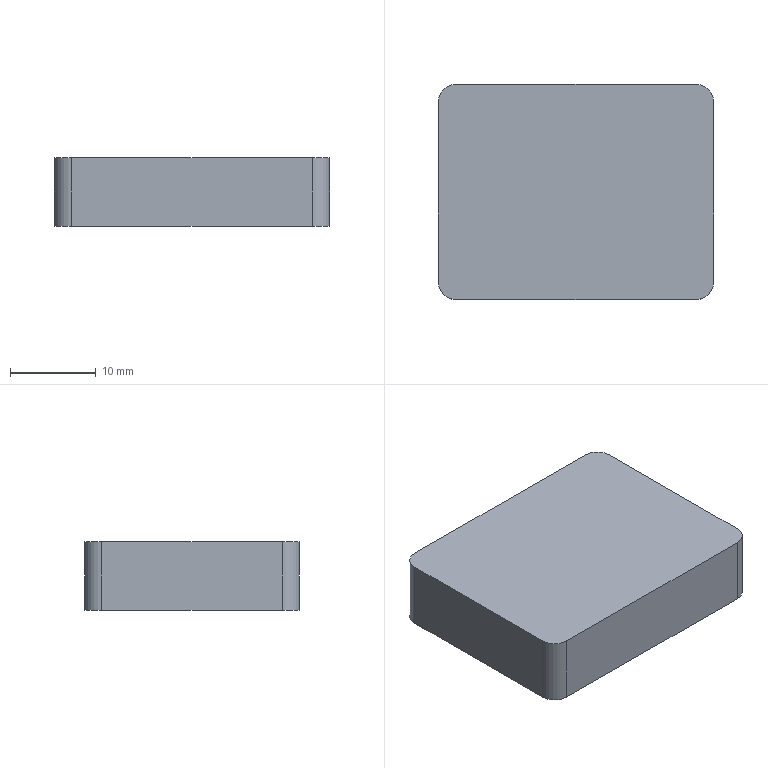CAM job | Mastercam | mm | 7 operations | part box 32 x 25 x 8
1. Facing | 24 - 100 平铣刀
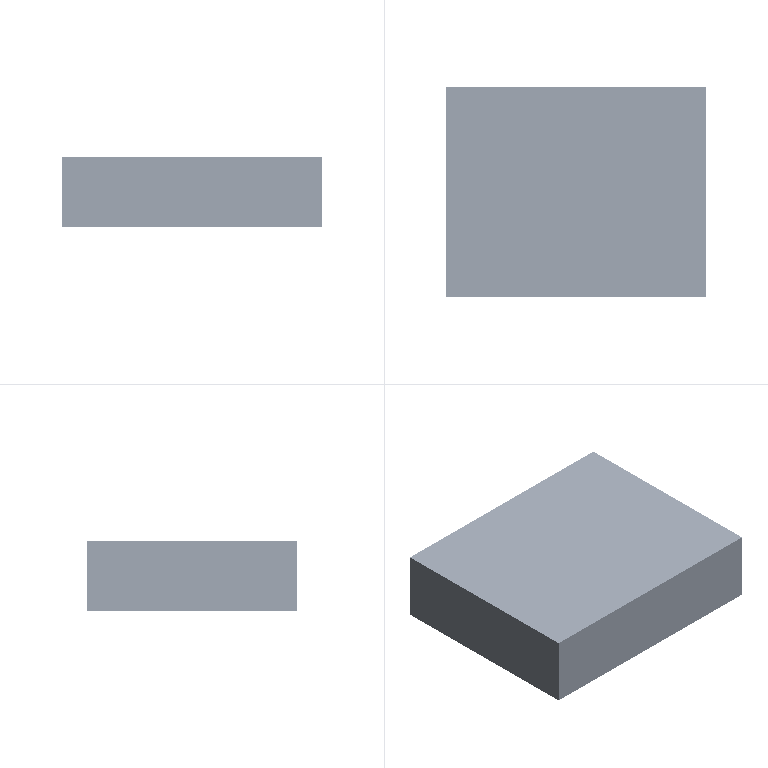2. Contour (Ramp) | 6 - 6 平铣刀
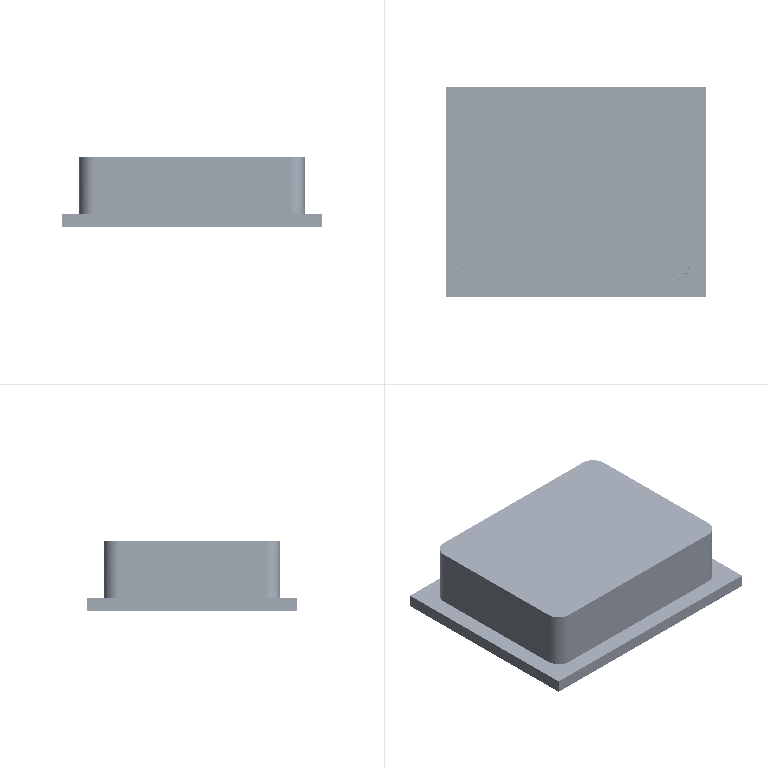3. Contour (Ramp) | 6 - 6 平铣刀
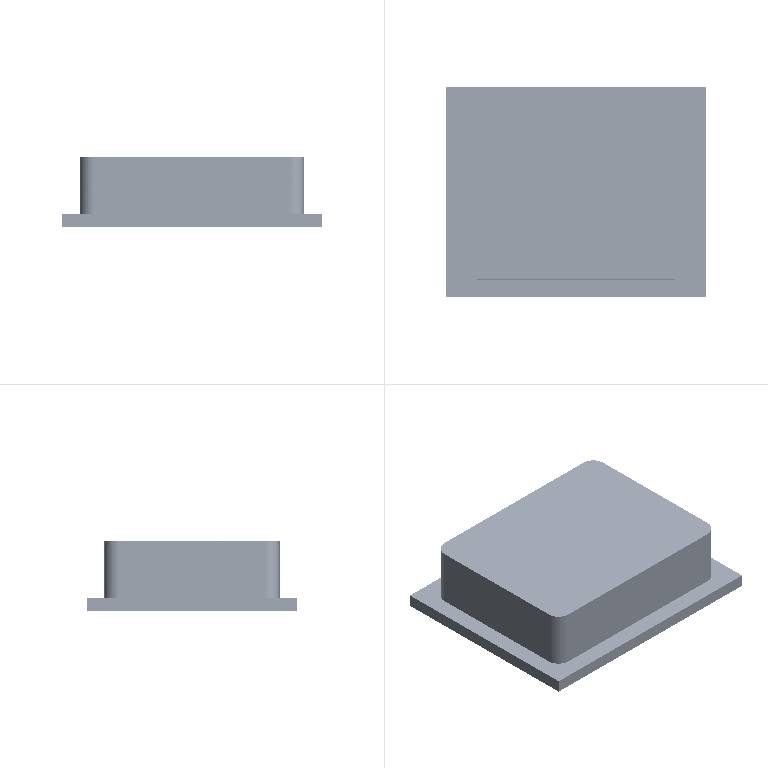4. Contour (2D chamfer) | 7 - 4 倒角刀
5. Facing | 24 - 100 平铣刀
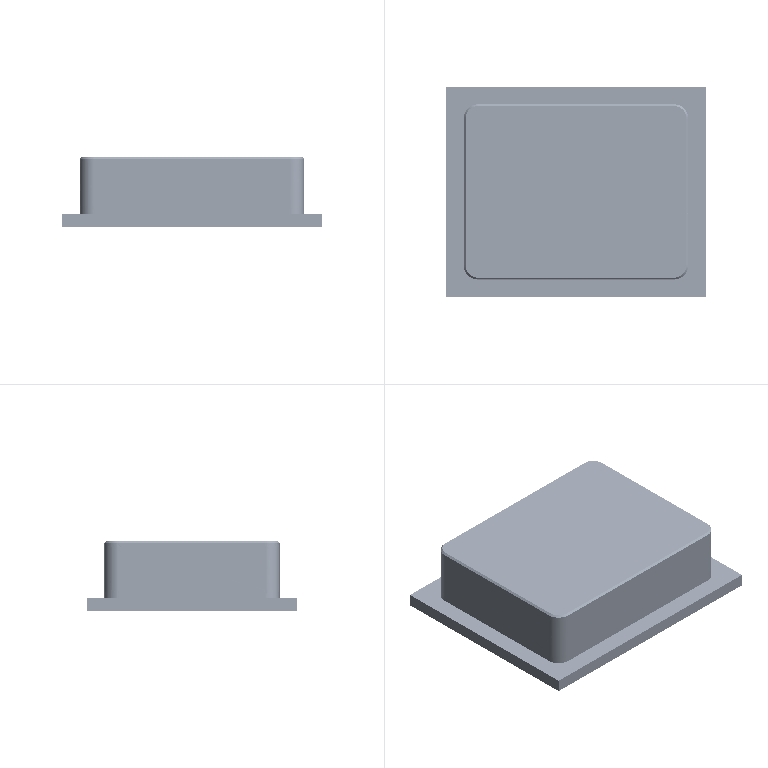6. Drill/Counterbore | 7 - 4 倒角刀
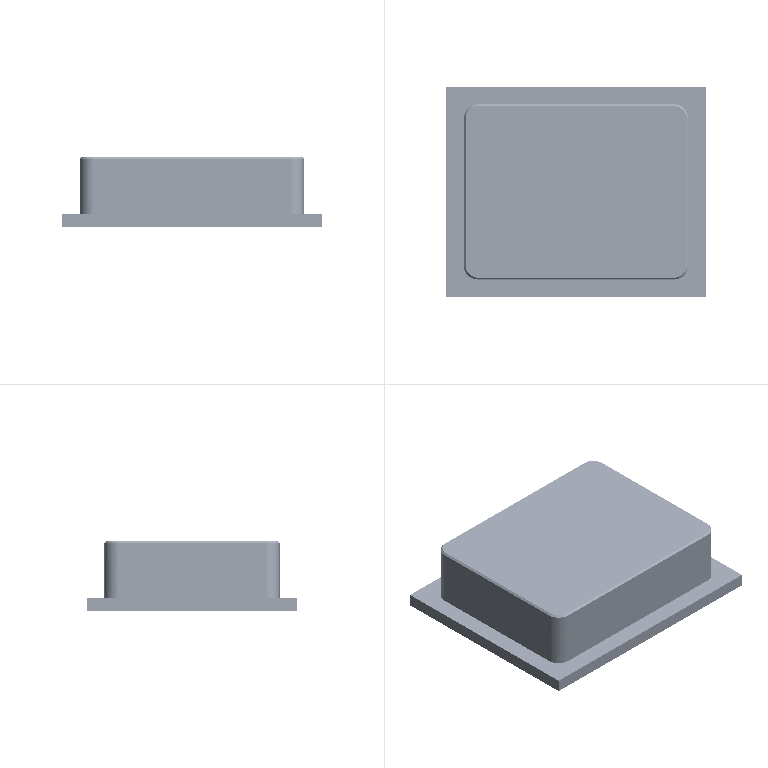7. Drill/Counterbore | 7 - 4 倒角刀